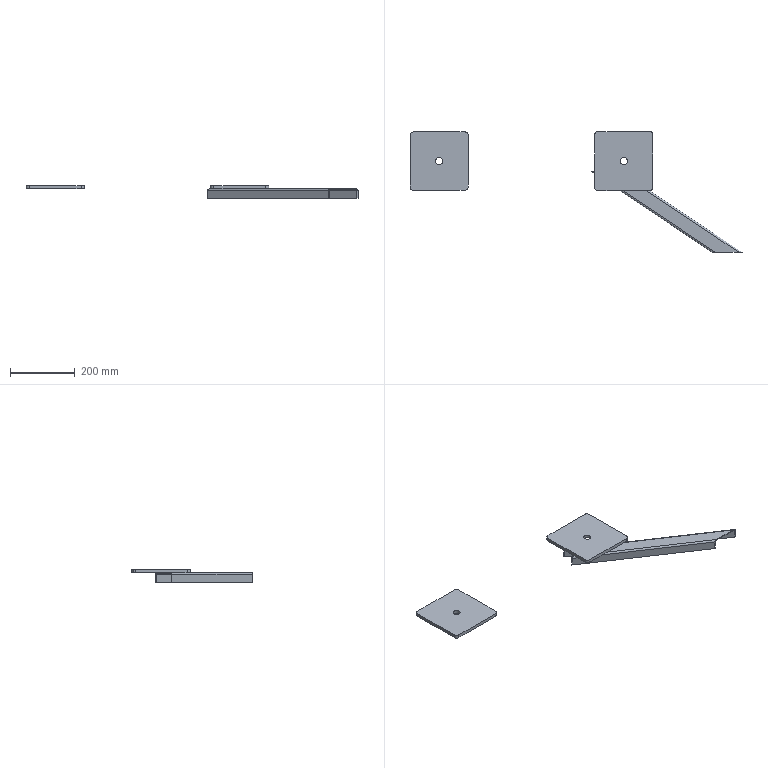Component | SolidWorks | 50x30x2ColdBentEqualAngleSteel550mmRight-1 | 3 solids | 41 faces | box 1024.97 x 373.11 x 40 mm | volume 743555 mm3 | plane 23 | cylinder 18 | commonest cylinder face diameters 20 x10 22 x4 10 x2 6 x2
build123d program:
from build123d import *

# Parameters (mm, degrees)
BOSS_EXTRUDE1_DEPTH     = 550
CUT_EXTRUDE1_2_DEPTH    = 88
CUT_EXTRUDE2_2_DEPTH    = 88
BOSS_EXTRUDE2_DEPTH     = 10
FILLET1_R               = 10
BOSS_EXTRUDE3_DEPTH     = 10
FILLET2_R               = 10
CUT_EXTRUDE1_DEPTH      = 648.638
CUT_EXTRUDE1_DEPTH_BACK = 648.638
SKETCH2_R               = 11
CUT_EXTRUDE2_DEPTH      = 5.01
SKETCH3_R               = 11
CUT_EXTRUDE3_DEPTH      = 5.01


with BuildPart() as part:
    # Sketch1_2 → Boss-Extrude1 (new body)
    with BuildSketch(Plane(origin=(0, 0, 0), x_dir=(0, 0, -1), z_dir=(1, 0, 0))):
        with BuildLine():
            Line((0, 5), (0, 45))
            ThreePointArc((0, 45), (1.464, 48.536), (5, 50))
            Line((5, 50), (30, 50))
            Line((30, 50), (30, 48))
            Line((30, 48), (5, 48))
            ThreePointArc((5, 48), (2.879, 47.121), (2, 45))
            Line((2, 45), (2, 5))
            ThreePointArc((2, 5), (2.879, 2.879), (5, 2))
            Line((5, 2), (30, 2))
            Line((30, 2), (30, 0))
            Line((30, 0), (5, 0))
            ThreePointArc((5, 0), (1.464, 1.464), (0, 5))
        make_face()
    extrude(amount=BOSS_EXTRUDE1_DEPTH)

    # Sketch2_2 → Cut-Extrude1_2 (cut)
    with BuildSketch(Plane.XY):
        Polygon((0, 50), (27.735, 8.397), (3.816, -7.548), (0, 0), align=None)
    extrude(amount=-CUT_EXTRUDE1_2_DEPTH, mode=Mode.SUBTRACT)

    # Sketch3_2 → Cut-Extrude2_2 (cut)
    with BuildSketch(Plane.XY):
        Polygon((540.833, 50), (488.532, 15.133), (518.711, -30.136), (550, 0), (550, 50), align=None)
    extrude(amount=-CUT_EXTRUDE2_2_DEPTH, mode=Mode.SUBTRACT)

    # Sketch1 → Cut-Extrude1 (cut, two sides: drawn at the far end of the back side and taken through both)
    with BuildSketch(Plane.XY.offset(-CUT_EXTRUDE1_DEPTH_BACK)):
        Polygon((481.566, -42.512), (573.092, 18.505), (548.618, 55.215), (457.093, -5.802), align=None)
    extrude(amount=CUT_EXTRUDE1_DEPTH + CUT_EXTRUDE1_DEPTH_BACK, mode=Mode.SUBTRACT)


with BuildPart() as body_2:
    # Sketch4 → Boss-Extrude2 (new body)
    with BuildSketch(Plane.XY):
        Polygon((105.045, 207.919), (-44.724, 108.073), (56.373, -43.573), (206.142, 56.273), align=None)
    extrude(amount=BOSS_EXTRUDE2_DEPTH)

    # Fillet1
    fillet1_edges = [body_2.edges().sort_by_distance(p)[0] for p in [
        (206.142, 56.273, 5),
        (56.373, -43.573, 5),
        (-44.724, 108.073, 5),
        (105.045, 207.919, 5),
    ]]
    fillet(fillet1_edges, radius=FILLET1_R)

    # Sketch2 → Cut-Extrude2 (cut, symmetric)
    with BuildSketch(Plane.XY.offset(5)):
        with Locations(Location((80.709, 82.173, 0), (0, 0, 180))):
            Circle(SKETCH2_R)
    extrude(amount=CUT_EXTRUDE2_DEPTH, both=True, mode=Mode.SUBTRACT)


with BuildPart() as body_3:
    # Sketch5 → Boss-Extrude3 (new body)
    with BuildSketch(Plane.XY):
        Polygon((-418.476, -358.882), (-268.707, -259.036), (-368.553, -109.267), (-518.322, -209.113), align=None)
    extrude(amount=BOSS_EXTRUDE3_DEPTH)

    # Fillet2
    fillet2_edges = [body_3.edges().sort_by_distance(p)[0] for p in [
        (-518.322, -209.113, 5),
        (-368.553, -109.267, 5),
        (-268.707, -259.036, 5),
        (-418.476, -358.882, 5),
    ]]
    fillet(fillet2_edges, radius=FILLET2_R)

    # Sketch3 → Cut-Extrude3 (cut, symmetric)
    with BuildSketch(Plane.XY.offset(5)):
        with Locations(Location((-393.56, -234.006, 0), (0, 0, 180))):
            Circle(SKETCH3_R)
    extrude(amount=CUT_EXTRUDE3_DEPTH, both=True, mode=Mode.SUBTRACT)


solid = Compound([part.part, body_2.part, body_3.part])

# Placed as in the assembly
solid = solid.moved(Location((197.894, 10.497, 415), (0, 0, -33.69)))